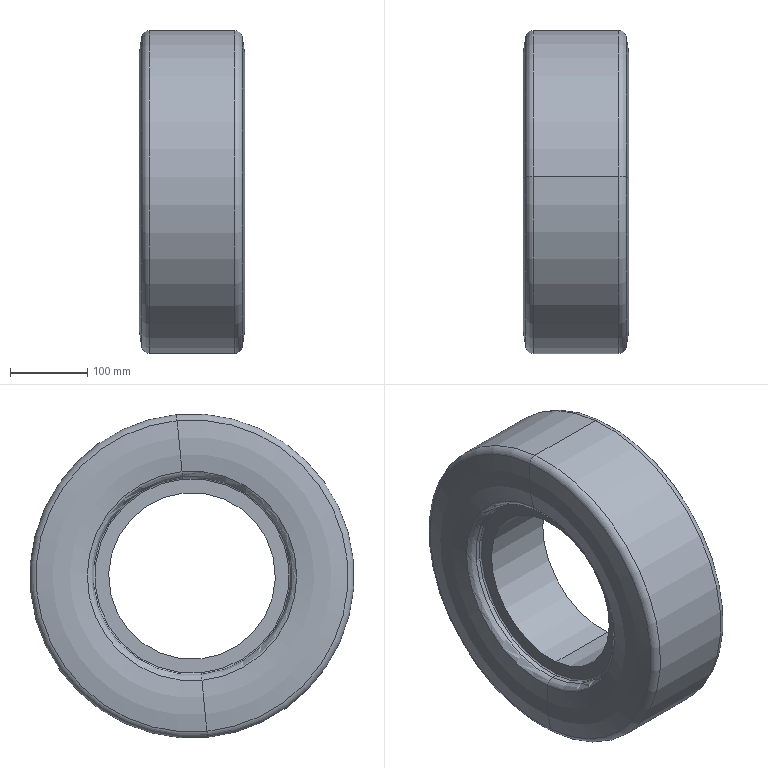Component | SolidWorks | Tire-1 | 1 solid | 26 faces | box 137.42 x 420 x 420 mm | volume 12981568 mm3 | torus 16 | cylinder 8 | plane 2 | commonest cylinder face diameters 256 x4 420 x2 216 x2
build123d program:
from build123d import *


with BuildPart() as part:
    # Sketch1 → Revolve2 (revolve)
    with BuildSketch(Plane.XY, mode=Mode.PRIVATE) as revolve2_sk:
        with BuildLine():
            Line((-47, 7.517), (-47, 25.517))
            ThreePointArc((-47, 25.517), (-47.586, 26.931), (-49, 27.517))
            Line((-49, 27.517), (-54.702, 27.517))
            Line((-54.702, 27.517), (-55.237, 27.517))
            ThreePointArc((-55.237, 27.517), (-61.476, 29.702), (-64.989, 35.303))
            ThreePointArc((-64.989, 35.303), (-68.712, 68.517), (-64.989, 101.731))
            ThreePointArc((-64.989, 101.731), (-61.476, 107.332), (-55.237, 109.517))
            Line((-55.237, 109.517), (55.237, 109.517))
            ThreePointArc((55.237, 109.517), (61.476, 107.332), (64.989, 101.731))
            ThreePointArc((64.989, 101.731), (68.712, 68.517), (64.989, 35.303))
            ThreePointArc((64.989, 35.303), (61.476, 29.702), (55.237, 27.517))
            Line((55.237, 27.517), (54.702, 27.517))
            Line((54.702, 27.517), (49, 27.517))
            ThreePointArc((49, 27.517), (47.586, 26.931), (47, 25.517))
            Line((47, 25.517), (47, 7.517))
            Line((47, 7.517), (-47, 7.517))
        make_face()
    revolve(revolve2_sk.sketch.rotate(Axis((-103.455, -100.483, 0), (1, 0, 0)), 90), axis=Axis((-103.455, -100.483, 0), (1, 0, 0)))


solid = part.part

# Placed as in the assembly
solid = solid.moved(Location((-561.371, -990.417, 148), (0, 0, 0)))
STEP:
#1=CARTESIAN_POINT('',(-23.952,-43.421,0.8887));
#2=VERTEX_POINT('',#1);
#3=CARTESIAN_POINT('',(-23.952,-42.476,10.765));
#4=VERTEX_POINT('',#3);
#5=CARTESIAN_POINT('',(-23.952,-42.949,5.827));
#6=DIRECTION('',(-1.,0.,-0.));
#7=DIRECTION('',(0.,0.09527,0.9955));
#8=AXIS2_PLACEMENT_3D('',#5,#6,#7);
#9=CIRCLE('',#8,4.961);
#10=EDGE_CURVE('',#2,#4,#9,.T.);
#11=ORIENTED_EDGE('',*,*,#10,.F.);
#12=CARTESIAN_POINT('',(-24.03,-43.429,0.8103));
#13=VERTEX_POINT('',#12);
#14=CARTESIAN_POINT('',(-24.03,-43.421,0.8887));
#15=DIRECTION('',(0.,0.9955,-0.09527));
#16=DIRECTION('',(0.,0.09527,0.9955));
#17=AXIS2_PLACEMENT_3D('',#14,#15,#16);
#18=CIRCLE('',#17,0.07874);
#19=EDGE_CURVE('',#2,#13,#18,.T.);
#20=ORIENTED_EDGE('',*,*,#19,.T.);
#21=CARTESIAN_POINT('',(-24.03,-42.469,10.843));
#22=VERTEX_POINT('',#21);
#23=CARTESIAN_POINT('',(-24.03,-42.949,5.827));
#24=DIRECTION('',(-1.,0.,-0.));
#25=DIRECTION('',(0.,0.09527,0.9955));
#26=AXIS2_PLACEMENT_3D('',#23,#24,#25);
#27=CIRCLE('',#26,5.039);
#28=EDGE_CURVE('',#13,#22,#27,.T.);
#29=ORIENTED_EDGE('',*,*,#28,.T.);
#30=CARTESIAN_POINT('',(-24.03,-42.476,10.765));
#31=DIRECTION('',(-0.,-0.9955,0.09527));
#32=DIRECTION('',(0.,-0.09527,-0.9955));
#33=AXIS2_PLACEMENT_3D('',#30,#31,#32);
#34=CIRCLE('',#33,0.07874);
#35=EDGE_CURVE('',#4,#22,#34,.T.);
#36=ORIENTED_EDGE('',*,*,#35,.F.);
#37=EDGE_LOOP('',(#11,#20,#29,#36));
#38=FACE_OUTER_BOUND('',#37,.T.);
#39=CARTESIAN_POINT('',(-24.03,-42.949,5.827));
#40=DIRECTION('',(-1.,0.,-0.));
#41=DIRECTION('',(-0.,0.09527,0.9955));
#42=AXIS2_PLACEMENT_3D('',#39,#40,#41);
#43=TOROIDAL_SURFACE('',#42,4.961,0.07874);
#44=ADVANCED_FACE('',(#38),#43,.F.);
#45=ORIENTED_EDGE('',*,*,#28,.F.);
#46=CARTESIAN_POINT('',(-24.276,-43.429,0.8103));
#47=VERTEX_POINT('',#46);
#48=CARTESIAN_POINT('',(-26.174,-43.429,0.8103));
#49=DIRECTION('',(-1.,0.,-0.));
#50=VECTOR('',#49,39.37);
#51=LINE('',#48,#50);
#52=EDGE_CURVE('',#13,#47,#51,.T.);
#53=ORIENTED_EDGE('',*,*,#52,.T.);
#54=CARTESIAN_POINT('',(-24.276,-42.469,10.843));
#55=VERTEX_POINT('',#54);
#56=CARTESIAN_POINT('',(-24.276,-42.949,5.827));
#57=DIRECTION('',(-1.,0.,-0.));
#58=DIRECTION('',(0.,0.09527,0.9955));
#59=AXIS2_PLACEMENT_3D('',#56,#57,#58);
#60=CIRCLE('',#59,5.039);
#61=EDGE_CURVE('',#47,#55,#60,.T.);
#62=ORIENTED_EDGE('',*,*,#61,.T.);
#63=CARTESIAN_POINT('',(-26.174,-42.469,10.843));
#64=DIRECTION('',(-1.,0.,-0.));
#65=VECTOR('',#64,39.37);
#66=LINE('',#63,#65);
#67=EDGE_CURVE('',#22,#55,#66,.T.);
#68=ORIENTED_EDGE('',*,*,#67,.F.);
#69=EDGE_LOOP('',(#45,#53,#62,#68));
#70=FACE_OUTER_BOUND('',#69,.T.);
#71=CARTESIAN_POINT('',(-26.174,-42.949,5.827));
#72=DIRECTION('',(-1.,0.,-0.));
#73=DIRECTION('',(0.,0.09527,0.9955));
#74=AXIS2_PLACEMENT_3D('',#71,#72,#73);
#75=CYLINDRICAL_SURFACE('',#74,5.039);
#76=ADVANCED_FACE('',(#70),#75,.F.);
#77=CARTESIAN_POINT('',(-24.66,-42.44,11.148));
#78=VERTEX_POINT('',#77);
#79=CARTESIAN_POINT('',(-24.66,-43.458,0.5052));
#80=VERTEX_POINT('',#79);
#81=CARTESIAN_POINT('',(-24.66,-42.949,5.827));
#82=DIRECTION('',(-1.,0.,-0.));
#83=DIRECTION('',(0.,0.09527,0.9955));
#84=AXIS2_PLACEMENT_3D('',#81,#82,#83);
#85=CIRCLE('',#84,5.346);
#86=EDGE_CURVE('',#78,#80,#85,.T.);
#87=ORIENTED_EDGE('',*,*,#86,.T.);
#88=CARTESIAN_POINT('',(-24.276,-43.466,0.4184));
#89=DIRECTION('',(0.,0.9955,-0.09527));
#90=DIRECTION('',(0.,0.09527,0.9955));
#91=AXIS2_PLACEMENT_3D('',#88,#89,#90);
#92=CIRCLE('',#91,0.3937);
#93=EDGE_CURVE('',#80,#47,#92,.T.);
#94=ORIENTED_EDGE('',*,*,#93,.T.);
#95=CARTESIAN_POINT('',(-24.276,-42.949,5.827));
#96=DIRECTION('',(-1.,0.,-0.));
#97=DIRECTION('',(0.,0.09527,0.9955));
#98=AXIS2_PLACEMENT_3D('',#95,#96,#97);
#99=CIRCLE('',#98,5.039);
#100=EDGE_CURVE('',#55,#47,#99,.T.);
#101=ORIENTED_EDGE('',*,*,#100,.F.);
#102=CARTESIAN_POINT('',(-24.276,-42.431,11.235));
#103=DIRECTION('',(-0.,-0.9955,0.09527));
#104=DIRECTION('',(0.,-0.09527,-0.9955));
#105=AXIS2_PLACEMENT_3D('',#102,#103,#104);
#106=CIRCLE('',#105,0.3937);
#107=EDGE_CURVE('',#78,#55,#106,.T.);
#108=ORIENTED_EDGE('',*,*,#107,.F.);
#109=EDGE_LOOP('',(#87,#94,#101,#108));
#110=FACE_OUTER_BOUND('',#109,.T.);
#111=CARTESIAN_POINT('',(-24.276,-42.949,5.827));
#112=DIRECTION('',(-1.,0.,-0.));
#113=DIRECTION('',(-0.,0.09527,0.9955));
#114=AXIS2_PLACEMENT_3D('',#111,#112,#113);
#115=TOROIDAL_SURFACE('',#114,5.433,0.3937);
#116=ADVANCED_FACE('',(#110),#115,.T.);
#117=CARTESIAN_POINT('',(-24.66,-42.19,13.752));
#118=VERTEX_POINT('',#117);
#119=CARTESIAN_POINT('',(-24.66,-43.707,-2.098));
#120=VERTEX_POINT('',#119);
#121=CARTESIAN_POINT('',(-24.66,-42.949,5.827));
#122=DIRECTION('',(-1.,0.,-0.));
#123=DIRECTION('',(0.,0.09527,0.9955));
#124=AXIS2_PLACEMENT_3D('',#121,#122,#123);
#125=CIRCLE('',#124,7.961);
#126=EDGE_CURVE('',#118,#120,#125,.T.);
#127=ORIENTED_EDGE('',*,*,#126,.T.);
#128=CARTESIAN_POINT('',(-18.901,-43.583,-0.7965));
#129=DIRECTION('',(0.,0.9955,-0.09527));
#130=DIRECTION('',(0.,0.09527,0.9955));
#131=AXIS2_PLACEMENT_3D('',#128,#129,#130);
#132=CIRCLE('',#131,5.906);
#133=EDGE_CURVE('',#120,#80,#132,.T.);
#134=ORIENTED_EDGE('',*,*,#133,.T.);
#135=ORIENTED_EDGE('',*,*,#86,.F.);
#136=CARTESIAN_POINT('',(-18.901,-42.315,12.45));
#137=DIRECTION('',(-0.,-0.9955,0.09527));
#138=DIRECTION('',(0.,-0.09527,-0.9955));
#139=AXIS2_PLACEMENT_3D('',#136,#137,#138);
#140=CIRCLE('',#139,5.906);
#141=EDGE_CURVE('',#118,#78,#140,.T.);
#142=ORIENTED_EDGE('',*,*,#141,.F.);
#143=EDGE_LOOP('',(#127,#134,#135,#142));
#144=FACE_OUTER_BOUND('',#143,.T.);
#145=CARTESIAN_POINT('',(-18.901,-42.949,5.827));
#146=DIRECTION('',(-1.,0.,-0.));
#147=DIRECTION('',(-0.,0.09527,0.9955));
#148=AXIS2_PLACEMENT_3D('',#145,#146,#147);
#149=TOROIDAL_SURFACE('',#148,6.654,5.906);
#150=ADVANCED_FACE('',(#144),#149,.T.);
#151=CARTESIAN_POINT('',(-24.276,-42.161,14.057));
#152=VERTEX_POINT('',#151);
#153=CARTESIAN_POINT('',(-24.276,-43.736,-2.403));
#154=VERTEX_POINT('',#153);
#155=CARTESIAN_POINT('',(-24.276,-42.949,5.827));
#156=DIRECTION('',(-1.,0.,-0.));
#157=DIRECTION('',(0.,0.09527,0.9955));
#158=AXIS2_PLACEMENT_3D('',#155,#156,#157);
#159=CIRCLE('',#158,8.268);
#160=EDGE_CURVE('',#152,#154,#159,.T.);
#161=ORIENTED_EDGE('',*,*,#160,.T.);
#162=CARTESIAN_POINT('',(-24.276,-43.699,-2.011));
#163=DIRECTION('',(0.,0.9955,-0.09527));
#164=DIRECTION('',(0.,0.09527,0.9955));
#165=AXIS2_PLACEMENT_3D('',#162,#163,#164);
#166=CIRCLE('',#165,0.3937);
#167=EDGE_CURVE('',#154,#120,#166,.T.);
#168=ORIENTED_EDGE('',*,*,#167,.T.);
#169=ORIENTED_EDGE('',*,*,#126,.F.);
#170=CARTESIAN_POINT('',(-24.276,-42.199,13.665));
#171=DIRECTION('',(-0.,-0.9955,0.09527));
#172=DIRECTION('',(0.,-0.09527,-0.9955));
#173=AXIS2_PLACEMENT_3D('',#170,#171,#172);
#174=CIRCLE('',#173,0.3937);
#175=EDGE_CURVE('',#152,#118,#174,.T.);
#176=ORIENTED_EDGE('',*,*,#175,.F.);
#177=EDGE_LOOP('',(#161,#168,#169,#176));
#178=FACE_OUTER_BOUND('',#177,.T.);
#179=CARTESIAN_POINT('',(-24.276,-42.949,5.827));
#180=DIRECTION('',(-1.,0.,-0.));
#181=DIRECTION('',(-0.,0.09527,0.9955));
#182=AXIS2_PLACEMENT_3D('',#179,#180,#181);
#183=TOROIDAL_SURFACE('',#182,7.874,0.3937);
#184=ADVANCED_FACE('',(#178),#183,.T.);
#185=CARTESIAN_POINT('',(-19.927,-42.161,14.057));
#186=VERTEX_POINT('',#185);
#187=CARTESIAN_POINT('',(-19.927,-43.736,-2.403));
#188=VERTEX_POINT('',#187);
#189=CARTESIAN_POINT('',(-19.927,-42.949,5.827));
#190=DIRECTION('',(-1.,0.,-0.));
#191=DIRECTION('',(0.,0.09527,0.9955));
#192=AXIS2_PLACEMENT_3D('',#189,#190,#191);
#193=CIRCLE('',#192,8.268);
#194=EDGE_CURVE('',#186,#188,#193,.T.);
#195=ORIENTED_EDGE('',*,*,#194,.T.);
#196=CARTESIAN_POINT('',(-26.174,-43.736,-2.403));
#197=DIRECTION('',(-1.,0.,-0.));
#198=VECTOR('',#197,39.37);
#199=LINE('',#196,#198);
#200=EDGE_CURVE('',#188,#154,#199,.T.);
#201=ORIENTED_EDGE('',*,*,#200,.T.);
#202=ORIENTED_EDGE('',*,*,#160,.F.);
#203=CARTESIAN_POINT('',(-26.174,-42.161,14.057));
#204=DIRECTION('',(-1.,0.,-0.));
#205=VECTOR('',#204,39.37);
#206=LINE('',#203,#205);
#207=EDGE_CURVE('',#186,#152,#206,.T.);
#208=ORIENTED_EDGE('',*,*,#207,.F.);
#209=EDGE_LOOP('',(#195,#201,#202,#208));
#210=FACE_OUTER_BOUND('',#209,.T.);
#211=CARTESIAN_POINT('',(-26.174,-42.949,5.827));
#212=DIRECTION('',(-1.,0.,-0.));
#213=DIRECTION('',(0.,0.09527,0.9955));
#214=AXIS2_PLACEMENT_3D('',#211,#212,#213);
#215=CYLINDRICAL_SURFACE('',#214,8.268);
#216=ADVANCED_FACE('',(#210),#215,.T.);
#217=CARTESIAN_POINT('',(-19.543,-42.19,13.752));
#218=VERTEX_POINT('',#217);
#219=CARTESIAN_POINT('',(-19.543,-43.707,-2.098));
#220=VERTEX_POINT('',#219);
#221=CARTESIAN_POINT('',(-19.543,-42.949,5.827));
#222=DIRECTION('',(-1.,0.,-0.));
#223=DIRECTION('',(0.,0.09527,0.9955));
#224=AXIS2_PLACEMENT_3D('',#221,#222,#223);
#225=CIRCLE('',#224,7.961);
#226=EDGE_CURVE('',#218,#220,#225,.T.);
#227=ORIENTED_EDGE('',*,*,#226,.T.);
#228=CARTESIAN_POINT('',(-19.927,-43.699,-2.011));
#229=DIRECTION('',(0.,0.9955,-0.09527));
#230=DIRECTION('',(0.,0.09527,0.9955));
#231=AXIS2_PLACEMENT_3D('',#228,#229,#230);
#232=CIRCLE('',#231,0.3937);
#233=EDGE_CURVE('',#220,#188,#232,.T.);
#234=ORIENTED_EDGE('',*,*,#233,.T.);
#235=ORIENTED_EDGE('',*,*,#194,.F.);
#236=CARTESIAN_POINT('',(-19.927,-42.199,13.665));
#237=DIRECTION('',(-0.,-0.9955,0.09527));
#238=DIRECTION('',(0.,-0.09527,-0.9955));
#239=AXIS2_PLACEMENT_3D('',#236,#237,#238);
#240=CIRCLE('',#239,0.3937);
#241=EDGE_CURVE('',#218,#186,#240,.T.);
#242=ORIENTED_EDGE('',*,*,#241,.F.);
#243=EDGE_LOOP('',(#227,#234,#235,#242));
#244=FACE_OUTER_BOUND('',#243,.T.);
#245=CARTESIAN_POINT('',(-19.927,-42.949,5.827));
#246=DIRECTION('',(-1.,0.,-0.));
#247=DIRECTION('',(-0.,0.09527,0.9955));
#248=AXIS2_PLACEMENT_3D('',#245,#246,#247);
#249=TOROIDAL_SURFACE('',#248,7.874,0.3937);
#250=ADVANCED_FACE('',(#244),#249,.T.);
#251=CARTESIAN_POINT('',(-19.543,-42.44,11.148));
#252=VERTEX_POINT('',#251);
#253=CARTESIAN_POINT('',(-19.543,-43.458,0.5052));
#254=VERTEX_POINT('',#253);
#255=CARTESIAN_POINT('',(-19.543,-42.949,5.827));
#256=DIRECTION('',(-1.,0.,-0.));
#257=DIRECTION('',(0.,0.09527,0.9955));
#258=AXIS2_PLACEMENT_3D('',#255,#256,#257);
#259=CIRCLE('',#258,5.346);
#260=EDGE_CURVE('',#252,#254,#259,.T.);
#261=ORIENTED_EDGE('',*,*,#260,.T.);
#262=CARTESIAN_POINT('',(-25.302,-43.583,-0.7965));
#263=DIRECTION('',(0.,0.9955,-0.09527));
#264=DIRECTION('',(0.,0.09527,0.9955));
#265=AXIS2_PLACEMENT_3D('',#262,#263,#264);
#266=CIRCLE('',#265,5.906);
#267=EDGE_CURVE('',#254,#220,#266,.T.);
#268=ORIENTED_EDGE('',*,*,#267,.T.);
#269=ORIENTED_EDGE('',*,*,#226,.F.);
#270=CARTESIAN_POINT('',(-25.302,-42.315,12.45));
#271=DIRECTION('',(-0.,-0.9955,0.09527));
#272=DIRECTION('',(0.,-0.09527,-0.9955));
#273=AXIS2_PLACEMENT_3D('',#270,#271,#272);
#274=CIRCLE('',#273,5.906);
#275=EDGE_CURVE('',#252,#218,#274,.T.);
#276=ORIENTED_EDGE('',*,*,#275,.F.);
#277=EDGE_LOOP('',(#261,#268,#269,#276));
#278=FACE_OUTER_BOUND('',#277,.T.);
#279=CARTESIAN_POINT('',(-25.302,-42.949,5.827));
#280=DIRECTION('',(-1.,0.,-0.));
#281=DIRECTION('',(-0.,0.09527,0.9955));
#282=AXIS2_PLACEMENT_3D('',#279,#280,#281);
#283=TOROIDAL_SURFACE('',#282,6.654,5.906);
#284=ADVANCED_FACE('',(#278),#283,.T.);
#285=CARTESIAN_POINT('',(-19.927,-42.469,10.843));
#286=VERTEX_POINT('',#285);
#287=CARTESIAN_POINT('',(-19.927,-43.429,0.8103));
#288=VERTEX_POINT('',#287);
#289=CARTESIAN_POINT('',(-19.927,-42.949,5.827));
#290=DIRECTION('',(-1.,0.,-0.));
#291=DIRECTION('',(0.,0.09527,0.9955));
#292=AXIS2_PLACEMENT_3D('',#289,#290,#291);
#293=CIRCLE('',#292,5.039);
#294=EDGE_CURVE('',#286,#288,#293,.T.);
#295=ORIENTED_EDGE('',*,*,#294,.T.);
#296=CARTESIAN_POINT('',(-19.927,-43.466,0.4184));
#297=DIRECTION('',(0.,0.9955,-0.09527));
#298=DIRECTION('',(0.,0.09527,0.9955));
#299=AXIS2_PLACEMENT_3D('',#296,#297,#298);
#300=CIRCLE('',#299,0.3937);
#301=EDGE_CURVE('',#288,#254,#300,.T.);
#302=ORIENTED_EDGE('',*,*,#301,.T.);
#303=ORIENTED_EDGE('',*,*,#260,.F.);
#304=CARTESIAN_POINT('',(-19.927,-42.431,11.235));
#305=DIRECTION('',(-0.,-0.9955,0.09527));
#306=DIRECTION('',(0.,-0.09527,-0.9955));
#307=AXIS2_PLACEMENT_3D('',#304,#305,#306);
#308=CIRCLE('',#307,0.3937);
#309=EDGE_CURVE('',#286,#252,#308,.T.);
#310=ORIENTED_EDGE('',*,*,#309,.F.);
#311=EDGE_LOOP('',(#295,#302,#303,#310));
#312=FACE_OUTER_BOUND('',#311,.T.);
#313=CARTESIAN_POINT('',(-19.927,-42.949,5.827));
#314=DIRECTION('',(-1.,0.,-0.));
#315=DIRECTION('',(-0.,0.09527,0.9955));
#316=AXIS2_PLACEMENT_3D('',#313,#314,#315);
#317=TOROIDAL_SURFACE('',#316,5.433,0.3937);
#318=ADVANCED_FACE('',(#312),#317,.T.);
#319=CARTESIAN_POINT('',(-19.927,-42.949,5.827));
#320=DIRECTION('',(-1.,0.,-0.));
#321=DIRECTION('',(0.,0.09527,0.9955));
#322=AXIS2_PLACEMENT_3D('',#319,#320,#321);
#323=CIRCLE('',#322,5.039);
#324=EDGE_CURVE('',#288,#286,#323,.T.);
#325=ORIENTED_EDGE('',*,*,#324,.F.);
#326=CARTESIAN_POINT('',(-20.172,-43.429,0.8103));
#327=VERTEX_POINT('',#326);
#328=CARTESIAN_POINT('',(-26.174,-43.429,0.8103));
#329=DIRECTION('',(-1.,0.,-0.));
#330=VECTOR('',#329,39.37);
#331=LINE('',#328,#330);
#332=EDGE_CURVE('',#288,#327,#331,.T.);
#333=ORIENTED_EDGE('',*,*,#332,.T.);
#334=CARTESIAN_POINT('',(-20.172,-42.469,10.843));
#335=VERTEX_POINT('',#334);
#336=CARTESIAN_POINT('',(-20.172,-42.949,5.827));
#337=DIRECTION('',(-1.,0.,-0.));
#338=DIRECTION('',(0.,0.09527,0.9955));
#339=AXIS2_PLACEMENT_3D('',#336,#337,#338);
#340=CIRCLE('',#339,5.039);
#341=EDGE_CURVE('',#327,#335,#340,.T.);
#342=ORIENTED_EDGE('',*,*,#341,.T.);
#343=CARTESIAN_POINT('',(-26.174,-42.469,10.843));
#344=DIRECTION('',(-1.,0.,-0.));
#345=VECTOR('',#344,39.37);
#346=LINE('',#343,#345);
#347=EDGE_CURVE('',#286,#335,#346,.T.);
#348=ORIENTED_EDGE('',*,*,#347,.F.);
#349=EDGE_LOOP('',(#325,#333,#342,#348));
#350=FACE_OUTER_BOUND('',#349,.T.);
#351=CARTESIAN_POINT('',(-26.174,-42.949,5.827));
#352=DIRECTION('',(-1.,0.,-0.));
#353=DIRECTION('',(0.,0.09527,0.9955));
#354=AXIS2_PLACEMENT_3D('',#351,#352,#353);
#355=CYLINDRICAL_SURFACE('',#354,5.039);
#356=ADVANCED_FACE('',(#350),#355,.F.);
#357=ORIENTED_EDGE('',*,*,#341,.F.);
#358=CARTESIAN_POINT('',(-20.251,-43.421,0.8887));
#359=VERTEX_POINT('',#358);
#360=CARTESIAN_POINT('',(-20.172,-43.421,0.8887));
#361=DIRECTION('',(0.,0.9955,-0.09527));
#362=DIRECTION('',(0.,0.09527,0.9955));
#363=AXIS2_PLACEMENT_3D('',#360,#361,#362);
#364=CIRCLE('',#363,0.07874);
#365=EDGE_CURVE('',#327,#359,#364,.T.);
#366=ORIENTED_EDGE('',*,*,#365,.T.);
#367=CARTESIAN_POINT('',(-20.251,-42.476,10.765));
#368=VERTEX_POINT('',#367);
#369=CARTESIAN_POINT('',(-20.251,-42.949,5.827));
#370=DIRECTION('',(-1.,0.,-0.));
#371=DIRECTION('',(0.,0.09527,0.9955));
#372=AXIS2_PLACEMENT_3D('',#369,#370,#371);
#373=CIRCLE('',#372,4.961);
#374=EDGE_CURVE('',#359,#368,#373,.T.);
#375=ORIENTED_EDGE('',*,*,#374,.T.);
#376=CARTESIAN_POINT('',(-20.172,-42.476,10.765));
#377=DIRECTION('',(-0.,-0.9955,0.09527));
#378=DIRECTION('',(0.,-0.09527,-0.9955));
#379=AXIS2_PLACEMENT_3D('',#376,#377,#378);
#380=CIRCLE('',#379,0.07874);
#381=EDGE_CURVE('',#335,#368,#380,.T.);
#382=ORIENTED_EDGE('',*,*,#381,.F.);
#383=EDGE_LOOP('',(#357,#366,#375,#382));
#384=FACE_OUTER_BOUND('',#383,.T.);
#385=CARTESIAN_POINT('',(-20.172,-42.949,5.827));
#386=DIRECTION('',(-1.,0.,-0.));
#387=DIRECTION('',(-0.,0.09527,0.9955));
#388=AXIS2_PLACEMENT_3D('',#385,#386,#387);
#389=TOROIDAL_SURFACE('',#388,4.961,0.07874);
#390=ADVANCED_FACE('',(#384),#389,.F.);
#391=CARTESIAN_POINT('',(-20.251,-43.354,1.594));
#392=VERTEX_POINT('',#391);
#393=CARTESIAN_POINT('',(-20.251,-42.544,10.059));
#394=VERTEX_POINT('',#393);
#395=CARTESIAN_POINT('',(-20.251,-42.949,5.827));
#396=DIRECTION('',(-1.,0.,-0.));
#397=DIRECTION('',(0.,0.09527,0.9955));
#398=AXIS2_PLACEMENT_3D('',#395,#396,#397);
#399=CIRCLE('',#398,4.252);
#400=EDGE_CURVE('',#392,#394,#399,.T.);
#401=ORIENTED_EDGE('',*,*,#400,.F.);
#402=CARTESIAN_POINT('',(-23.952,-43.354,1.594));
#403=VERTEX_POINT('',#402);
#404=CARTESIAN_POINT('',(-26.174,-43.354,1.594));
#405=DIRECTION('',(-1.,0.,-0.));
#406=VECTOR('',#405,39.37);
#407=LINE('',#404,#406);
#408=EDGE_CURVE('',#392,#403,#407,.T.);
#409=ORIENTED_EDGE('',*,*,#408,.T.);
#410=CARTESIAN_POINT('',(-23.952,-42.544,10.059));
#411=VERTEX_POINT('',#410);
#412=CARTESIAN_POINT('',(-23.952,-42.949,5.827));
#413=DIRECTION('',(-1.,0.,-0.));
#414=DIRECTION('',(0.,0.09527,0.9955));
#415=AXIS2_PLACEMENT_3D('',#412,#413,#414);
#416=CIRCLE('',#415,4.252);
#417=EDGE_CURVE('',#403,#411,#416,.T.);
#418=ORIENTED_EDGE('',*,*,#417,.T.);
#419=CARTESIAN_POINT('',(-26.174,-42.544,10.059));
#420=DIRECTION('',(-1.,0.,-0.));
#421=VECTOR('',#420,39.37);
#422=LINE('',#419,#421);
#423=EDGE_CURVE('',#394,#411,#422,.T.);
#424=ORIENTED_EDGE('',*,*,#423,.F.);
#425=EDGE_LOOP('',(#401,#409,#418,#424));
#426=FACE_OUTER_BOUND('',#425,.T.);
#427=CARTESIAN_POINT('',(-26.174,-42.949,5.827));
#428=DIRECTION('',(-1.,0.,-0.));
#429=DIRECTION('',(0.,0.09527,0.9955));
#430=AXIS2_PLACEMENT_3D('',#427,#428,#429);
#431=CYLINDRICAL_SURFACE('',#430,4.252);
#432=ADVANCED_FACE('',(#426),#431,.F.);
#433=ORIENTED_EDGE('',*,*,#408,.F.);
#434=CARTESIAN_POINT('',(-20.251,-42.949,5.827));
#435=DIRECTION('',(-1.,0.,-0.));
#436=DIRECTION('',(0.,0.09527,0.9955));
#437=AXIS2_PLACEMENT_3D('',#434,#435,#436);
#438=CIRCLE('',#437,4.252);
#439=EDGE_CURVE('',#394,#392,#438,.T.);
#440=ORIENTED_EDGE('',*,*,#439,.F.);
#441=ORIENTED_EDGE('',*,*,#423,.T.);
#442=CARTESIAN_POINT('',(-23.952,-42.949,5.827));
#443=DIRECTION('',(-1.,0.,-0.));
#444=DIRECTION('',(0.,0.09527,0.9955));
#445=AXIS2_PLACEMENT_3D('',#442,#443,#444);
#446=CIRCLE('',#445,4.252);
#447=EDGE_CURVE('',#411,#403,#446,.T.);
#448=ORIENTED_EDGE('',*,*,#447,.T.);
#449=EDGE_LOOP('',(#433,#440,#441,#448));
#450=FACE_OUTER_BOUND('',#449,.T.);
#451=CARTESIAN_POINT('',(-26.174,-42.949,5.827));
#452=DIRECTION('',(-1.,0.,-0.));
#453=DIRECTION('',(0.,0.09527,0.9955));
#454=AXIS2_PLACEMENT_3D('',#451,#452,#453);
#455=CYLINDRICAL_SURFACE('',#454,4.252);
#456=ADVANCED_FACE('',(#450),#455,.F.);
#457=CARTESIAN_POINT('',(-20.251,-42.949,5.827));
#458=DIRECTION('',(-1.,0.,-0.));
#459=DIRECTION('',(0.,0.09527,0.9955));
#460=AXIS2_PLACEMENT_3D('',#457,#458,#459);
#461=CIRCLE('',#460,4.961);
#462=EDGE_CURVE('',#368,#359,#461,.T.);
#463=ORIENTED_EDGE('',*,*,#462,.F.);
#464=ORIENTED_EDGE('',*,*,#374,.F.);
#465=EDGE_LOOP('',(#463,#464));
#466=FACE_OUTER_BOUND('',#465,.T.);
#467=ORIENTED_EDGE('',*,*,#439,.T.);
#468=ORIENTED_EDGE('',*,*,#400,.T.);
#469=EDGE_LOOP('',(#467,#468));
#470=FACE_BOUND('',#469,.T.);
#471=CARTESIAN_POINT('',(-20.251,-38.716,5.422));
#472=DIRECTION('',(-1.,0.,-0.));
#473=DIRECTION('',(-0.,0.09527,0.9955));
#474=AXIS2_PLACEMENT_3D('',#471,#472,#473);
#475=PLANE('',#474);
#476=ADVANCED_FACE('',(#466,#470),#475,.F.);
#477=ORIENTED_EDGE('',*,*,#365,.F.);
#478=CARTESIAN_POINT('',(-20.172,-42.949,5.827));
#479=DIRECTION('',(-1.,0.,-0.));
#480=DIRECTION('',(0.,0.09527,0.9955));
#481=AXIS2_PLACEMENT_3D('',#478,#479,#480);
#482=CIRCLE('',#481,5.039);
#483=EDGE_CURVE('',#335,#327,#482,.T.);
#484=ORIENTED_EDGE('',*,*,#483,.F.);
#485=ORIENTED_EDGE('',*,*,#381,.T.);
#486=ORIENTED_EDGE('',*,*,#462,.T.);
#487=EDGE_LOOP('',(#477,#484,#485,#486));
#488=FACE_OUTER_BOUND('',#487,.T.);
#489=CARTESIAN_POINT('',(-20.172,-42.949,5.827));
#490=DIRECTION('',(-1.,0.,-0.));
#491=DIRECTION('',(-0.,0.09527,0.9955));
#492=AXIS2_PLACEMENT_3D('',#489,#490,#491);
#493=TOROIDAL_SURFACE('',#492,4.961,0.07874);
#494=ADVANCED_FACE('',(#488),#493,.F.);
#495=ORIENTED_EDGE('',*,*,#332,.F.);
#496=ORIENTED_EDGE('',*,*,#294,.F.);
#497=ORIENTED_EDGE('',*,*,#347,.T.);
#498=ORIENTED_EDGE('',*,*,#483,.T.);
#499=EDGE_LOOP('',(#495,#496,#497,#498));
#500=FACE_OUTER_BOUND('',#499,.T.);
#501=CARTESIAN_POINT('',(-26.174,-42.949,5.827));
#502=DIRECTION('',(-1.,0.,-0.));
#503=DIRECTION('',(0.,0.09527,0.9955));
#504=AXIS2_PLACEMENT_3D('',#501,#502,#503);
#505=CYLINDRICAL_SURFACE('',#504,5.039);
#506=ADVANCED_FACE('',(#500),#505,.F.);
#507=ORIENTED_EDGE('',*,*,#301,.F.);
#508=ORIENTED_EDGE('',*,*,#324,.T.);
#509=ORIENTED_EDGE('',*,*,#309,.T.);
#510=CARTESIAN_POINT('',(-19.543,-42.949,5.827));
#511=DIRECTION('',(-1.,0.,-0.));
#512=DIRECTION('',(0.,0.09527,0.9955));
#513=AXIS2_PLACEMENT_3D('',#510,#511,#512);
#514=CIRCLE('',#513,5.346);
#515=EDGE_CURVE('',#254,#252,#514,.T.);
#516=ORIENTED_EDGE('',*,*,#515,.F.);
#517=EDGE_LOOP('',(#507,#508,#509,#516));
#518=FACE_OUTER_BOUND('',#517,.T.);
#519=CARTESIAN_POINT('',(-19.927,-42.949,5.827));
#520=DIRECTION('',(-1.,0.,-0.));
#521=DIRECTION('',(-0.,0.09527,0.9955));
#522=AXIS2_PLACEMENT_3D('',#519,#520,#521);
#523=TOROIDAL_SURFACE('',#522,5.433,0.3937);
#524=ADVANCED_FACE('',(#518),#523,.T.);
#525=ORIENTED_EDGE('',*,*,#267,.F.);
#526=ORIENTED_EDGE('',*,*,#515,.T.);
#527=ORIENTED_EDGE('',*,*,#275,.T.);
#528=CARTESIAN_POINT('',(-19.543,-42.949,5.827));
#529=DIRECTION('',(-1.,0.,-0.));
#530=DIRECTION('',(0.,0.09527,0.9955));
#531=AXIS2_PLACEMENT_3D('',#528,#529,#530);
#532=CIRCLE('',#531,7.961);
#533=EDGE_CURVE('',#220,#218,#532,.T.);
#534=ORIENTED_EDGE('',*,*,#533,.F.);
#535=EDGE_LOOP('',(#525,#526,#527,#534));
#536=FACE_OUTER_BOUND('',#535,.T.);
#537=CARTESIAN_POINT('',(-25.302,-42.949,5.827));
#538=DIRECTION('',(-1.,0.,-0.));
#539=DIRECTION('',(-0.,0.09527,0.9955));
#540=AXIS2_PLACEMENT_3D('',#537,#538,#539);
#541=TOROIDAL_SURFACE('',#540,6.654,5.906);
#542=ADVANCED_FACE('',(#536),#541,.T.);
#543=ORIENTED_EDGE('',*,*,#233,.F.);
#544=ORIENTED_EDGE('',*,*,#533,.T.);
#545=ORIENTED_EDGE('',*,*,#241,.T.);
#546=CARTESIAN_POINT('',(-19.927,-42.949,5.827));
#547=DIRECTION('',(-1.,0.,-0.));
#548=DIRECTION('',(0.,0.09527,0.9955));
#549=AXIS2_PLACEMENT_3D('',#546,#547,#548);
#550=CIRCLE('',#549,8.268);
#551=EDGE_CURVE('',#188,#186,#550,.T.);
#552=ORIENTED_EDGE('',*,*,#551,.F.);
#553=EDGE_LOOP('',(#543,#544,#545,#552));
#554=FACE_OUTER_BOUND('',#553,.T.);
#555=CARTESIAN_POINT('',(-19.927,-42.949,5.827));
#556=DIRECTION('',(-1.,0.,-0.));
#557=DIRECTION('',(-0.,0.09527,0.9955));
#558=AXIS2_PLACEMENT_3D('',#555,#556,#557);
#559=TOROIDAL_SURFACE('',#558,7.874,0.3937);
#560=ADVANCED_FACE('',(#554),#559,.T.);
#561=ORIENTED_EDGE('',*,*,#200,.F.);
#562=ORIENTED_EDGE('',*,*,#551,.T.);
#563=ORIENTED_EDGE('',*,*,#207,.T.);
#564=CARTESIAN_POINT('',(-24.276,-42.949,5.827));
#565=DIRECTION('',(-1.,0.,-0.));
#566=DIRECTION('',(0.,0.09527,0.9955));
#567=AXIS2_PLACEMENT_3D('',#564,#565,#566);
#568=CIRCLE('',#567,8.268);
#569=EDGE_CURVE('',#154,#152,#568,.T.);
#570=ORIENTED_EDGE('',*,*,#569,.F.);
#571=EDGE_LOOP('',(#561,#562,#563,#570));
#572=FACE_OUTER_BOUND('',#571,.T.);
#573=CARTESIAN_POINT('',(-26.174,-42.949,5.827));
#574=DIRECTION('',(-1.,0.,-0.));
#575=DIRECTION('',(0.,0.09527,0.9955));
#576=AXIS2_PLACEMENT_3D('',#573,#574,#575);
#577=CYLINDRICAL_SURFACE('',#576,8.268);
#578=ADVANCED_FACE('',(#572),#577,.T.);
#579=ORIENTED_EDGE('',*,*,#167,.F.);
#580=ORIENTED_EDGE('',*,*,#569,.T.);
#581=ORIENTED_EDGE('',*,*,#175,.T.);
#582=CARTESIAN_POINT('',(-24.66,-42.949,5.827));
#583=DIRECTION('',(-1.,0.,-0.));
#584=DIRECTION('',(0.,0.09527,0.9955));
#585=AXIS2_PLACEMENT_3D('',#582,#583,#584);
#586=CIRCLE('',#585,7.961);
#587=EDGE_CURVE('',#120,#118,#586,.T.);
#588=ORIENTED_EDGE('',*,*,#587,.F.);
#589=EDGE_LOOP('',(#579,#580,#581,#588));
#590=FACE_OUTER_BOUND('',#589,.T.);
#591=CARTESIAN_POINT('',(-24.276,-42.949,5.827));
#592=DIRECTION('',(-1.,0.,-0.));
#593=DIRECTION('',(-0.,0.09527,0.9955));
#594=AXIS2_PLACEMENT_3D('',#591,#592,#593);
#595=TOROIDAL_SURFACE('',#594,7.874,0.3937);
#596=ADVANCED_FACE('',(#590),#595,.T.);
#597=ORIENTED_EDGE('',*,*,#133,.F.);
#598=ORIENTED_EDGE('',*,*,#587,.T.);
#599=ORIENTED_EDGE('',*,*,#141,.T.);
#600=CARTESIAN_POINT('',(-24.66,-42.949,5.827));
#601=DIRECTION('',(-1.,0.,-0.));
#602=DIRECTION('',(0.,0.09527,0.9955));
#603=AXIS2_PLACEMENT_3D('',#600,#601,#602);
#604=CIRCLE('',#603,5.346);
#605=EDGE_CURVE('',#80,#78,#604,.T.);
#606=ORIENTED_EDGE('',*,*,#605,.F.);
#607=EDGE_LOOP('',(#597,#598,#599,#606));
#608=FACE_OUTER_BOUND('',#607,.T.);
#609=CARTESIAN_POINT('',(-18.901,-42.949,5.827));
#610=DIRECTION('',(-1.,0.,-0.));
#611=DIRECTION('',(-0.,0.09527,0.9955));
#612=AXIS2_PLACEMENT_3D('',#609,#610,#611);
#613=TOROIDAL_SURFACE('',#612,6.654,5.906);
#614=ADVANCED_FACE('',(#608),#613,.T.);
#615=ORIENTED_EDGE('',*,*,#93,.F.);
#616=ORIENTED_EDGE('',*,*,#605,.T.);
#617=ORIENTED_EDGE('',*,*,#107,.T.);
#618=ORIENTED_EDGE('',*,*,#61,.F.);
#619=EDGE_LOOP('',(#615,#616,#617,#618));
#620=FACE_OUTER_BOUND('',#619,.T.);
#621=CARTESIAN_POINT('',(-24.276,-42.949,5.827));
#622=DIRECTION('',(-1.,0.,-0.));
#623=DIRECTION('',(-0.,0.09527,0.9955));
#624=AXIS2_PLACEMENT_3D('',#621,#622,#623);
#625=TOROIDAL_SURFACE('',#624,5.433,0.3937);
#626=ADVANCED_FACE('',(#620),#625,.T.);
#627=ORIENTED_EDGE('',*,*,#52,.F.);
#628=CARTESIAN_POINT('',(-24.03,-42.949,5.827));
#629=DIRECTION('',(-1.,0.,-0.));
#630=DIRECTION('',(0.,0.09527,0.9955));
#631=AXIS2_PLACEMENT_3D('',#628,#629,#630);
#632=CIRCLE('',#631,5.039);
#633=EDGE_CURVE('',#22,#13,#632,.T.);
#634=ORIENTED_EDGE('',*,*,#633,.F.);
#635=ORIENTED_EDGE('',*,*,#67,.T.);
#636=ORIENTED_EDGE('',*,*,#100,.T.);
#637=EDGE_LOOP('',(#627,#634,#635,#636));
#638=FACE_OUTER_BOUND('',#637,.T.);
#639=CARTESIAN_POINT('',(-26.174,-42.949,5.827));
#640=DIRECTION('',(-1.,0.,-0.));
#641=DIRECTION('',(0.,0.09527,0.9955));
#642=AXIS2_PLACEMENT_3D('',#639,#640,#641);
#643=CYLINDRICAL_SURFACE('',#642,5.039);
#644=ADVANCED_FACE('',(#638),#643,.F.);
#645=ORIENTED_EDGE('',*,*,#19,.F.);
#646=CARTESIAN_POINT('',(-23.952,-42.949,5.827));
#647=DIRECTION('',(-1.,0.,-0.));
#648=DIRECTION('',(0.,0.09527,0.9955));
#649=AXIS2_PLACEMENT_3D('',#646,#647,#648);
#650=CIRCLE('',#649,4.961);
#651=EDGE_CURVE('',#4,#2,#650,.T.);
#652=ORIENTED_EDGE('',*,*,#651,.F.);
#653=ORIENTED_EDGE('',*,*,#35,.T.);
#654=ORIENTED_EDGE('',*,*,#633,.T.);
#655=EDGE_LOOP('',(#645,#652,#653,#654));
#656=FACE_OUTER_BOUND('',#655,.T.);
#657=CARTESIAN_POINT('',(-24.03,-42.949,5.827));
#658=DIRECTION('',(-1.,0.,-0.));
#659=DIRECTION('',(-0.,0.09527,0.9955));
#660=AXIS2_PLACEMENT_3D('',#657,#658,#659);
#661=TOROIDAL_SURFACE('',#660,4.961,0.07874);
#662=ADVANCED_FACE('',(#656),#661,.F.);
#663=ORIENTED_EDGE('',*,*,#447,.F.);
#664=ORIENTED_EDGE('',*,*,#417,.F.);
#665=EDGE_LOOP('',(#663,#664));
#666=FACE_BOUND('',#665,.T.);
#667=ORIENTED_EDGE('',*,*,#651,.T.);
#668=ORIENTED_EDGE('',*,*,#10,.T.);
#669=EDGE_LOOP('',(#667,#668));
#670=FACE_OUTER_BOUND('',#669,.T.);
#671=CARTESIAN_POINT('',(-23.952,-38.716,5.422));
#672=DIRECTION('',(1.,-0.,0.));
#673=DIRECTION('',(0.,-0.09527,-0.9955));
#674=AXIS2_PLACEMENT_3D('',#671,#672,#673);
#675=PLANE('',#674);
#676=ADVANCED_FACE('',(#666,#670),#675,.F.);
#677=CLOSED_SHELL('',(#44,#76,#116,#150,#184,#216,#250,#284,#318,#356,#390,#432,#456,#476,#494,#506,#524,#542,#560,#578,#596,#614,#626,#644,#662,#676));
#678=MANIFOLD_SOLID_BREP('',#677);
#679=CARTESIAN_POINT('',(0.,0.,0.));
#680=DIRECTION('',(0.,0.,1.));
#681=DIRECTION('',(1.,0.,0.));
#682=AXIS2_PLACEMENT_3D('',#679,#680,#681);
#683=(LENGTH_UNIT()NAMED_UNIT(*)SI_UNIT($,.METRE.));
#684=LENGTH_MEASURE_WITH_UNIT(LENGTH_MEASURE(0.0254),#683);
#685=DIMENSIONAL_EXPONENTS(1.,0.,0.,0.,0.,0.,0.);
#686=(CONVERSION_BASED_UNIT('',#684)LENGTH_UNIT()NAMED_UNIT(#685));
#687=UNCERTAINTY_MEASURE_WITH_UNIT(LENGTH_MEASURE(0.00001),#686,'','');
#688=(NAMED_UNIT(*)PLANE_ANGLE_UNIT()SI_UNIT($,.RADIAN.));
#689=(NAMED_UNIT(*)SI_UNIT($,.STERADIAN.)SOLID_ANGLE_UNIT());
#690=(GEOMETRIC_REPRESENTATION_CONTEXT(3)GLOBAL_UNCERTAINTY_ASSIGNED_CONTEXT((#687))GLOBAL_UNIT_ASSIGNED_CONTEXT((#686,#688,#689))REPRESENTATION_CONTEXT('',''));
#691=ADVANCED_BREP_SHAPE_REPRESENTATION('',(#678,#682),#690);
#692=COLOUR_RGB('',0.7922,0.8196,0.9333);
#693=FILL_AREA_STYLE_COLOUR('',#692);
#694=FILL_AREA_STYLE('',(#693));
#695=SURFACE_STYLE_FILL_AREA(#694);
#696=SURFACE_SIDE_STYLE('',(#695));
#697=SURFACE_STYLE_USAGE(.BOTH.,#696);
#698=PRESENTATION_STYLE_ASSIGNMENT((#697));
#699=STYLED_ITEM('',(#698),#678);
#700=PRESENTATION_LAYER_ASSIGNMENT('','',(#699));
#701=(LENGTH_UNIT()NAMED_UNIT(*)SI_UNIT($,.METRE.));
#702=LENGTH_MEASURE_WITH_UNIT(LENGTH_MEASURE(0.0254),#701);
#703=DIMENSIONAL_EXPONENTS(1.,0.,0.,0.,0.,0.,0.);
#704=(CONVERSION_BASED_UNIT('',#702)LENGTH_UNIT()NAMED_UNIT(#703));
#705=UNCERTAINTY_MEASURE_WITH_UNIT(LENGTH_MEASURE(0.00001),#704,'','');
#706=(NAMED_UNIT(*)PLANE_ANGLE_UNIT()SI_UNIT($,.RADIAN.));
#707=(NAMED_UNIT(*)SI_UNIT($,.STERADIAN.)SOLID_ANGLE_UNIT());
#708=(GEOMETRIC_REPRESENTATION_CONTEXT(3)GLOBAL_UNCERTAINTY_ASSIGNED_CONTEXT((#705))GLOBAL_UNIT_ASSIGNED_CONTEXT((#704,#706,#707))REPRESENTATION_CONTEXT('',''));
#709=MECHANICAL_DESIGN_GEOMETRIC_PRESENTATION_REPRESENTATION('',(#699),#708);